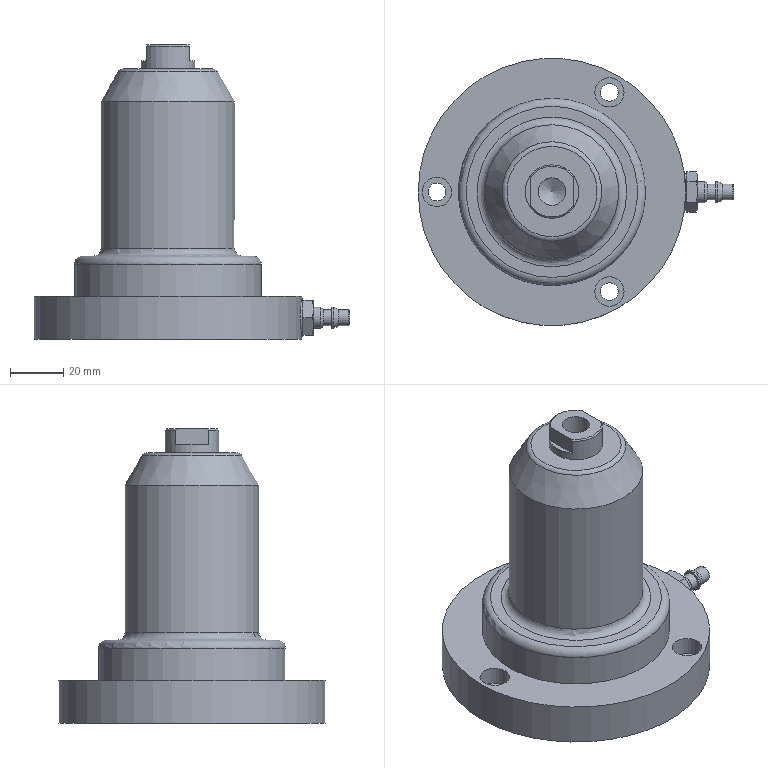Assembly | NX | mm | 14 component files | 14 solids | 229 faces | box 118 x 100 x 110 mm | volume 263749 mm3 | plane 111 | cylinder 66 | cone 32 | torus 15 | spline 5 | commonest cylinder face diameters 6 x14 11 x9 10 x7 40 x6 7 x6 6.6 x3 5 x2 9.728 x2
Bill of materials:
unnamed part 1 | 1 |  | Cylindrical helical coil of round-section wire with about 7-8 open turns. The end coils look closed and flattened, which resembles a compression spring.
unnamed part 2 | 1 |  | Long hollow cylindrical stem standing on a larger circular flange. The flange has a circumferential groove around its rim. The top end has an axial bore and what look like flats near the tip.
unnamed part 3 | 1 |  | Thin flat annular ring with a rectangular cross-section, like a thin washer or shim.
unnamed part 4 | 1 |  | Flanged cylindrical bushing with a through axial bore. The top end is chamfered or tapered, a short flange sits at the base, and a very small radial hole is visible on the side of the body.
unnamed part 5 | 1 |  | Annular ring with a rectangular cross-section, axially thicker than the other flat rings. Looks like a spacer or sleeve ring.
unnamed part 6 | 1 |  | Fitting-like body with a central hexagonal collar. A plain cylindrical shank extends on one side; on the other side is a stepped spigot with a tapered, barb-like ridge. A through bore runs along the axis.
unnamed part 7 | 1 |  | Flat annular ring with a fairly wide radial wall relative to its diameter and a rectangular cross-section, like a washer or spacer.
unnamed part 8 | 6 |  | Headed cylindrical pin or screw-like part: a plain cylindrical shank with a chamfered free end, on a larger short cylindrical head.
unnamed part 9 | 1 |  | Circular disc with a low raised central boss. The boss holds a shallow circular recess with a small countersunk center hole. The disc has a ring of axial through holes and one radial side port.
Mates:
1. fix | End_Cap 1 component
2. concentric | End_Cap_Seal 1 edge | Cylinder 1 edge
3. concentric | Cylinder 1 edge | End_Cap 1 edge
4. touch align | End_Cap 1 face | Cylinder 1 face
5. concentric | Piston_Seal 1 edge | Piston_Rod 1 edge
6. concentric | Spring 1 edge | Piston_Rod 1 edge
7. touch align | Piston_Seal 1 face | Cylinder 1 face
8. touch align | Spring 1 face | Cylinder 1 face
9. concentric | Tube_Seal 1 edge | Tube_Fitting 1 edge
10. concentric | Tube_Seal 1 edge | End_Cap 1 arc
11. concentric | Screw 6 edge | End_Cap 1 edge
12. bond | Cylinder 1 component | assembly component
13. bond | Screw 6 component | assembly component
14. bond | Screw 5 component | assembly component
15. bond | Screw 4 component | assembly component
16. bond | Screw 3 component | assembly component
17. circular | assembly datumaxis | assembly cartesiancoordinatesystem | assembly cartesiancoordinatesystem | assembly cartesiancoordinatesystem | assembly cartesiancoordinatesystem | assembly cartesiancoordinatesystem | assembly cartesiancoordinatesystem
18. bond | Screw 2 component | assembly component
19. bond | Screw 1 component | assembly component